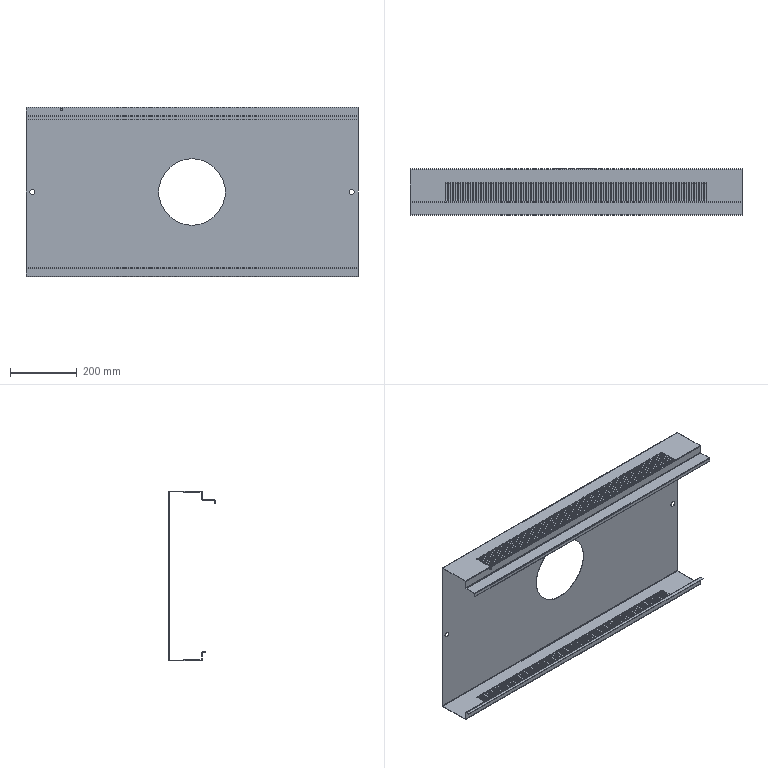Component | SolidWorks | AirFurnaceElectricalCabinet-TopPlate-2 | 1 solid | 2282 faces | volume 940173 mm3 | cylinder 1286 | plane 996 | commonest cylinder face diameters 6 x632 3.6 x316 8.4 x316 1.5 x7 3.9 x7 15.5 x4 6.5 x2 200 x2